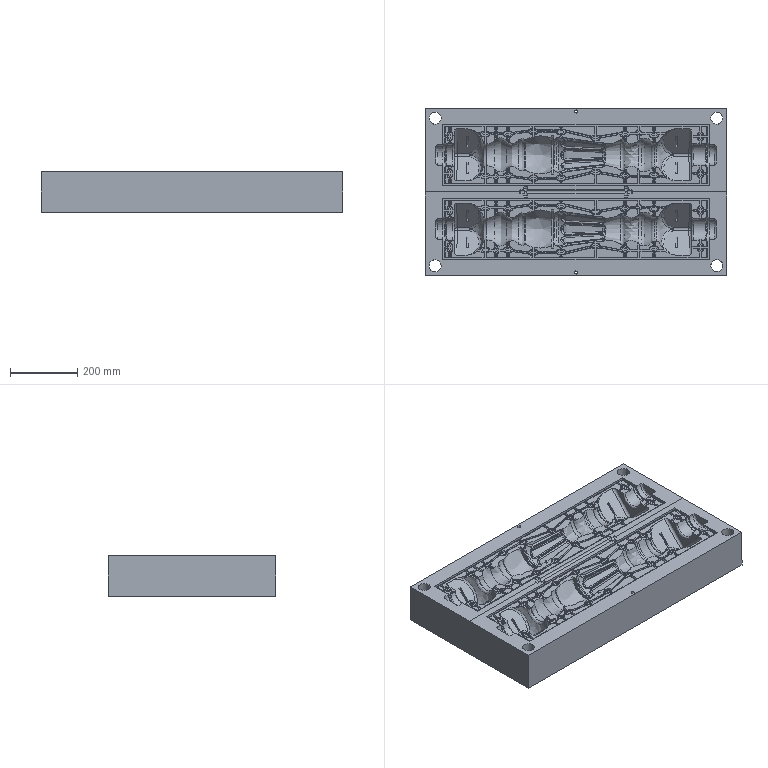CAM job | NX | mm | 3-axis | 1 set-up | 3 operations | part box 900 x 500 x 120
set-up 1
1. Cavity Milling | Mill Mill5 D30R5 | CAVITY_MILL_COPY | path 1457298.862 mm | 573.278 min
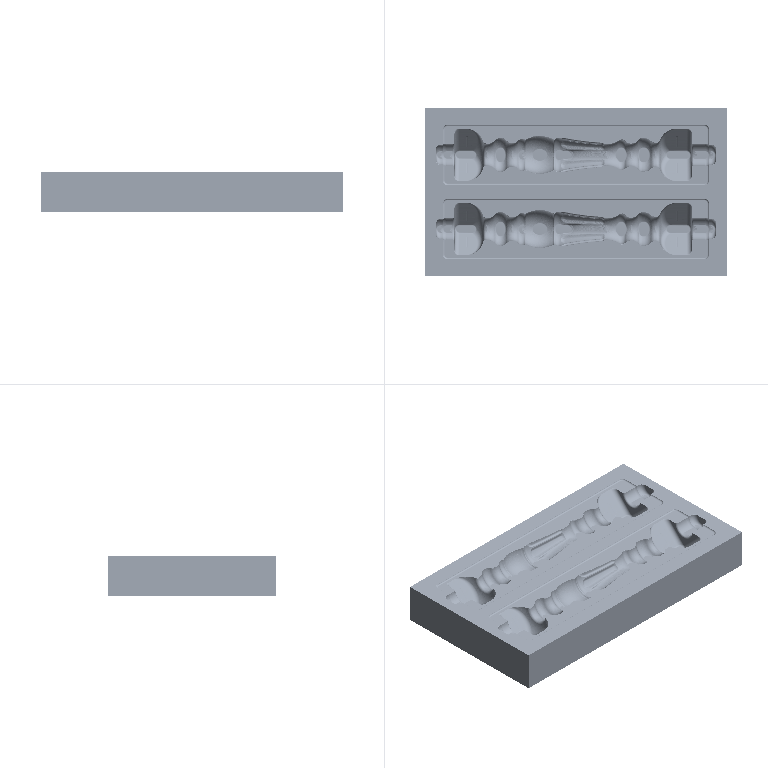2. Z-Level Milling | Mill Mill5 D10 | ZLEVEL_PROFILE_4 | path 32253.311 mm | 12.886 min
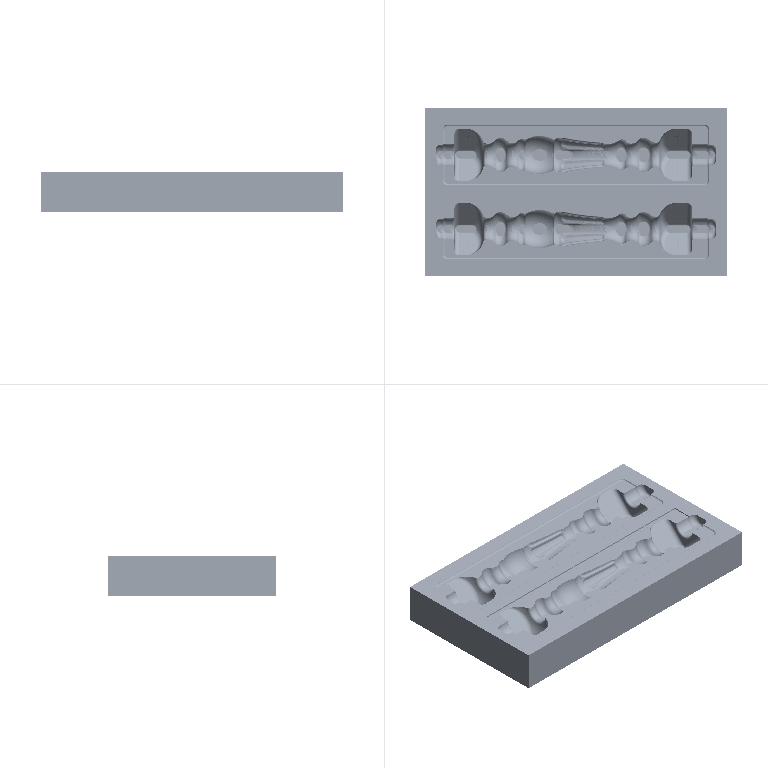3. Face Milling | Mill Mill5 D10 | FACE_MILLING_1 | path 6554.804 mm | 2.605 min